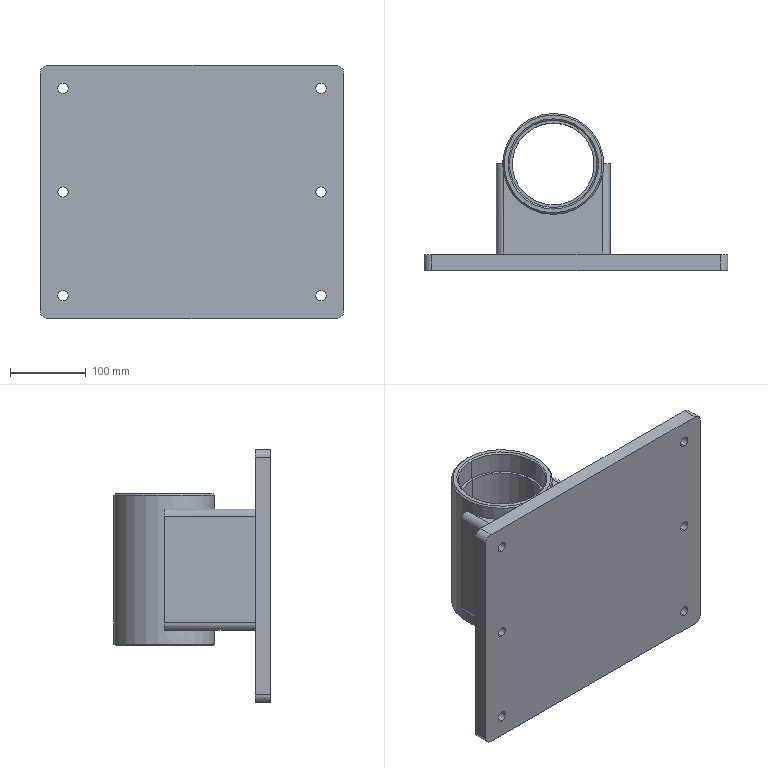Component | SolidWorks | CuttingMachineRotaryBase-1 | 2 solids | 61 faces | box 400 x 206.5 x 333.5 mm | volume 3801643 mm3 | cylinder 32 | plane 21 | cone 8 | commonest cylinder face diameters 13.5 x12 20 x8 115 x4 10 x4 108 x2 133 x2 | material Stainless Steel
build123d program:
from build123d import *

# Parameters (mm, degrees)
BOSS_EXTRUDE1_DEPTH      = 120
SKETCH2_R                = 66.5
CUT_EXTRUDE1_DEPTH       = 214.6
SKETCH3_W                = 333.5
SKETCH3_H                = 400
BOSS_EXTRUDE2_DEPTH      = 20
BOSS_EXTRUDE3_DEPTH      = 100
BOSS_EXTRUDE3_DEPTH_BACK = 100
SKETCH4_R                = 66.5
SKETCH4_R_2              = 57.5
FILLET1_R                = 10
SKETCH5_R                = 6.75
CUT_EXTRUDE2_DEPTH       = 20
SKETCH6_R                = 57.5
SKETCH6_R_2              = 54
BOSS_EXTRUDE4_DEPTH      = 140
CHAMFER1_SIZE            = 2


with BuildPart() as part:
    # Sketch1 → Boss-Extrude1 (new body)
    with BuildSketch(Plane.XY):
        with BuildLine():
            Line((70, -75), (-70, -75))
            ThreePointArc((-70, -75), (-77.071, -72.071), (-80, -65))
            Line((-80, -65), (-80, 65))
            ThreePointArc((-80, 65), (-77.071, 72.071), (-70, 75))
            Line((-70, 75), (70, 75))
            ThreePointArc((70, 75), (77.071, 72.071), (80, 65))
            Line((80, 65), (80, -65))
            ThreePointArc((80, -65), (77.071, -72.071), (70, -75))
        make_face()
        with BuildLine():
            Line((70, 70), (-70, 70))
            ThreePointArc((-70, 70), (-73.536, 68.536), (-75, 65))
            Line((-75, 65), (-75, -65))
            ThreePointArc((-75, -65), (-73.536, -68.536), (-70, -70))
            Line((-70, -70), (70, -70))
            ThreePointArc((70, -70), (73.536, -68.536), (75, -65))
            Line((75, -65), (75, 65))
            ThreePointArc((75, 65), (73.536, 68.536), (70, 70))
        make_face(mode=Mode.SUBTRACT)
    extrude(amount=BOSS_EXTRUDE1_DEPTH)

    # Sketch2 → Cut-Extrude1 (cut, through all)
    with BuildSketch(Plane.ZY.offset(80)):
        with Locations((120, 0)):
            Circle(SKETCH2_R)
    extrude(amount=-CUT_EXTRUDE1_DEPTH, mode=Mode.SUBTRACT)



with BuildPart() as body_2:
    # Sketch3 → Boss-Extrude2 (new body)
    with BuildSketch(Plane(origin=(0, 0, 0), x_dir=(-1, 0, 0), z_dir=(0, 0, -1))):
        with Locations((-8.25, -30)):
            Rectangle(SKETCH3_W, SKETCH3_H)
    extrude(amount=BOSS_EXTRUDE2_DEPTH)

    # Fillet1
    fillet1_edges = [body_2.edges().sort_by_distance(p)[0] for p in [
        (-158.5, -230, -10),
        (175, -230, -10),
        (175, 170, -10),
        (-158.5, 170, -10),
    ]]
    fillet(fillet1_edges, radius=FILLET1_R)

    # Sketch5 → Cut-Extrude2 (cut)
    with BuildSketch(Plane.XY):
        with Locations((-128.5, -200)):
            Circle(SKETCH5_R)
        with Locations((8.25, -200)):
            Circle(SKETCH5_R)
        with Locations((145, -200)):
            Circle(SKETCH5_R)
        with Locations((-128.5, 140)):
            Circle(SKETCH5_R)
        with Locations((8.25, 140)):
            Circle(SKETCH5_R)
        with Locations((145, 140)):
            Circle(SKETCH5_R)
    extrude(amount=-CUT_EXTRUDE2_DEPTH, mode=Mode.SUBTRACT)


with BuildPart() as body_3:
    # Sketch4 → Boss-Extrude3 (new, two sides: drawn at the far end of the back side and taken through both)
    with BuildSketch(Plane(origin=(0, 0, 0), x_dir=(0, 0, -1), z_dir=(1, 0, 0)).offset(-BOSS_EXTRUDE3_DEPTH_BACK)):
        with Locations((-120, 0)):
            Circle(SKETCH4_R)
        with Locations((-120, 0)):
            Circle(SKETCH4_R_2, mode=Mode.SUBTRACT)
    extrude(amount=BOSS_EXTRUDE3_DEPTH + BOSS_EXTRUDE3_DEPTH_BACK)


with BuildPart() as part_1:
    add(part.part)

    add(body_3.part)  # Boss-Extrude4 merges body 3
    # Sketch6 → Boss-Extrude4 (add)
    with BuildSketch(Plane.ZY.offset(70)):
        with Locations(Location((120, 0, 0), (0, 0, 180))):
            Circle(SKETCH6_R)
        with Locations((120, 0)):
            Circle(SKETCH6_R_2, mode=Mode.SUBTRACT)
    extrude(amount=-BOSS_EXTRUDE4_DEPTH)

    # Chamfer1
    chamfer1_edges = [part_1.edges().sort_by_distance(p)[0] for p in [
        (-100, 0, 186.5),
        (-100, 0, 177.5),
        (100, 0, 177.5),
        (100, 0, 186.5),
    ]]
    chamfer(chamfer1_edges, length=CHAMFER1_SIZE)


solid = Compound([body_2.part, part_1.part])

# Placed as in the assembly
solid = solid.moved(Location((-534.67, 847.452, 250.7), (-90, 0, 90)))